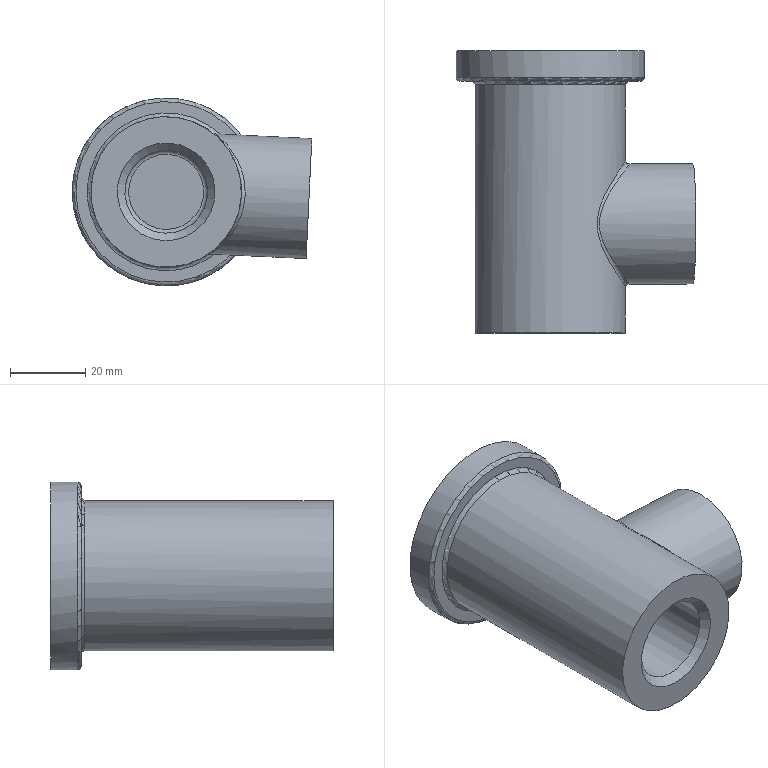Component | NX | HOUSING | 1 solid | 25 faces | volume 84245 mm3 | cylinder 8 | plane 8 | spline 4 | torus 3 | cone 2 | commonest cylinder face diameters 16 x1 40 x1 50 x1 32 x1 30 x1 22 x1 17 x1 10 x1